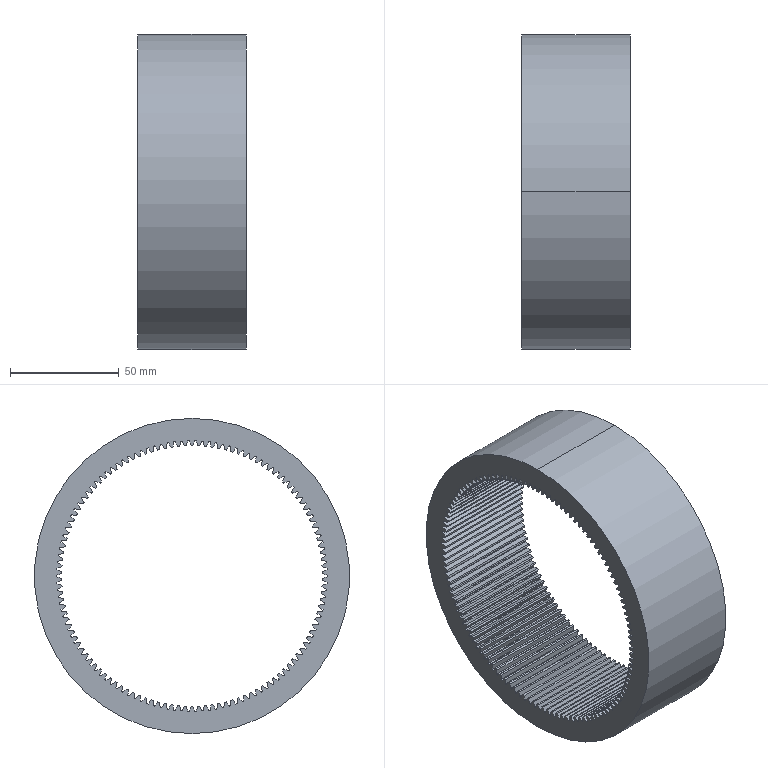Component | SolidWorks | 23RingGear-1 | 1 solid | 493 faces | volume 239864 mm3 | cylinder 247 | plane 246 | commonest cylinder face diameters 120 x123 124.5 x122 145 x2